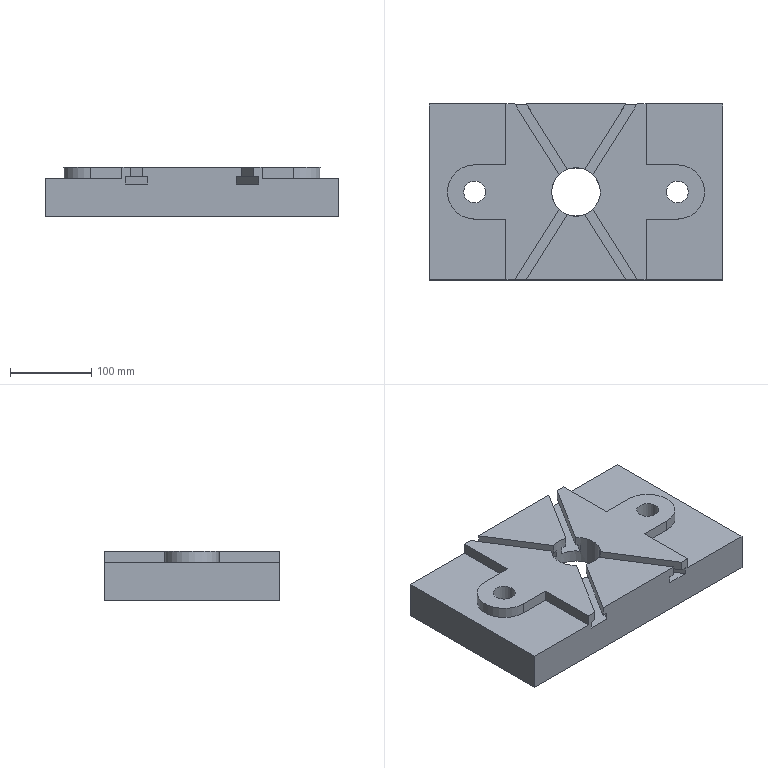Component | NX | BASE | 1 solid | 58 faces | volume 2647151 mm3 | plane 52 | cylinder 6 | commonest cylinder face diameters 67 x2 60 x2 27 x2